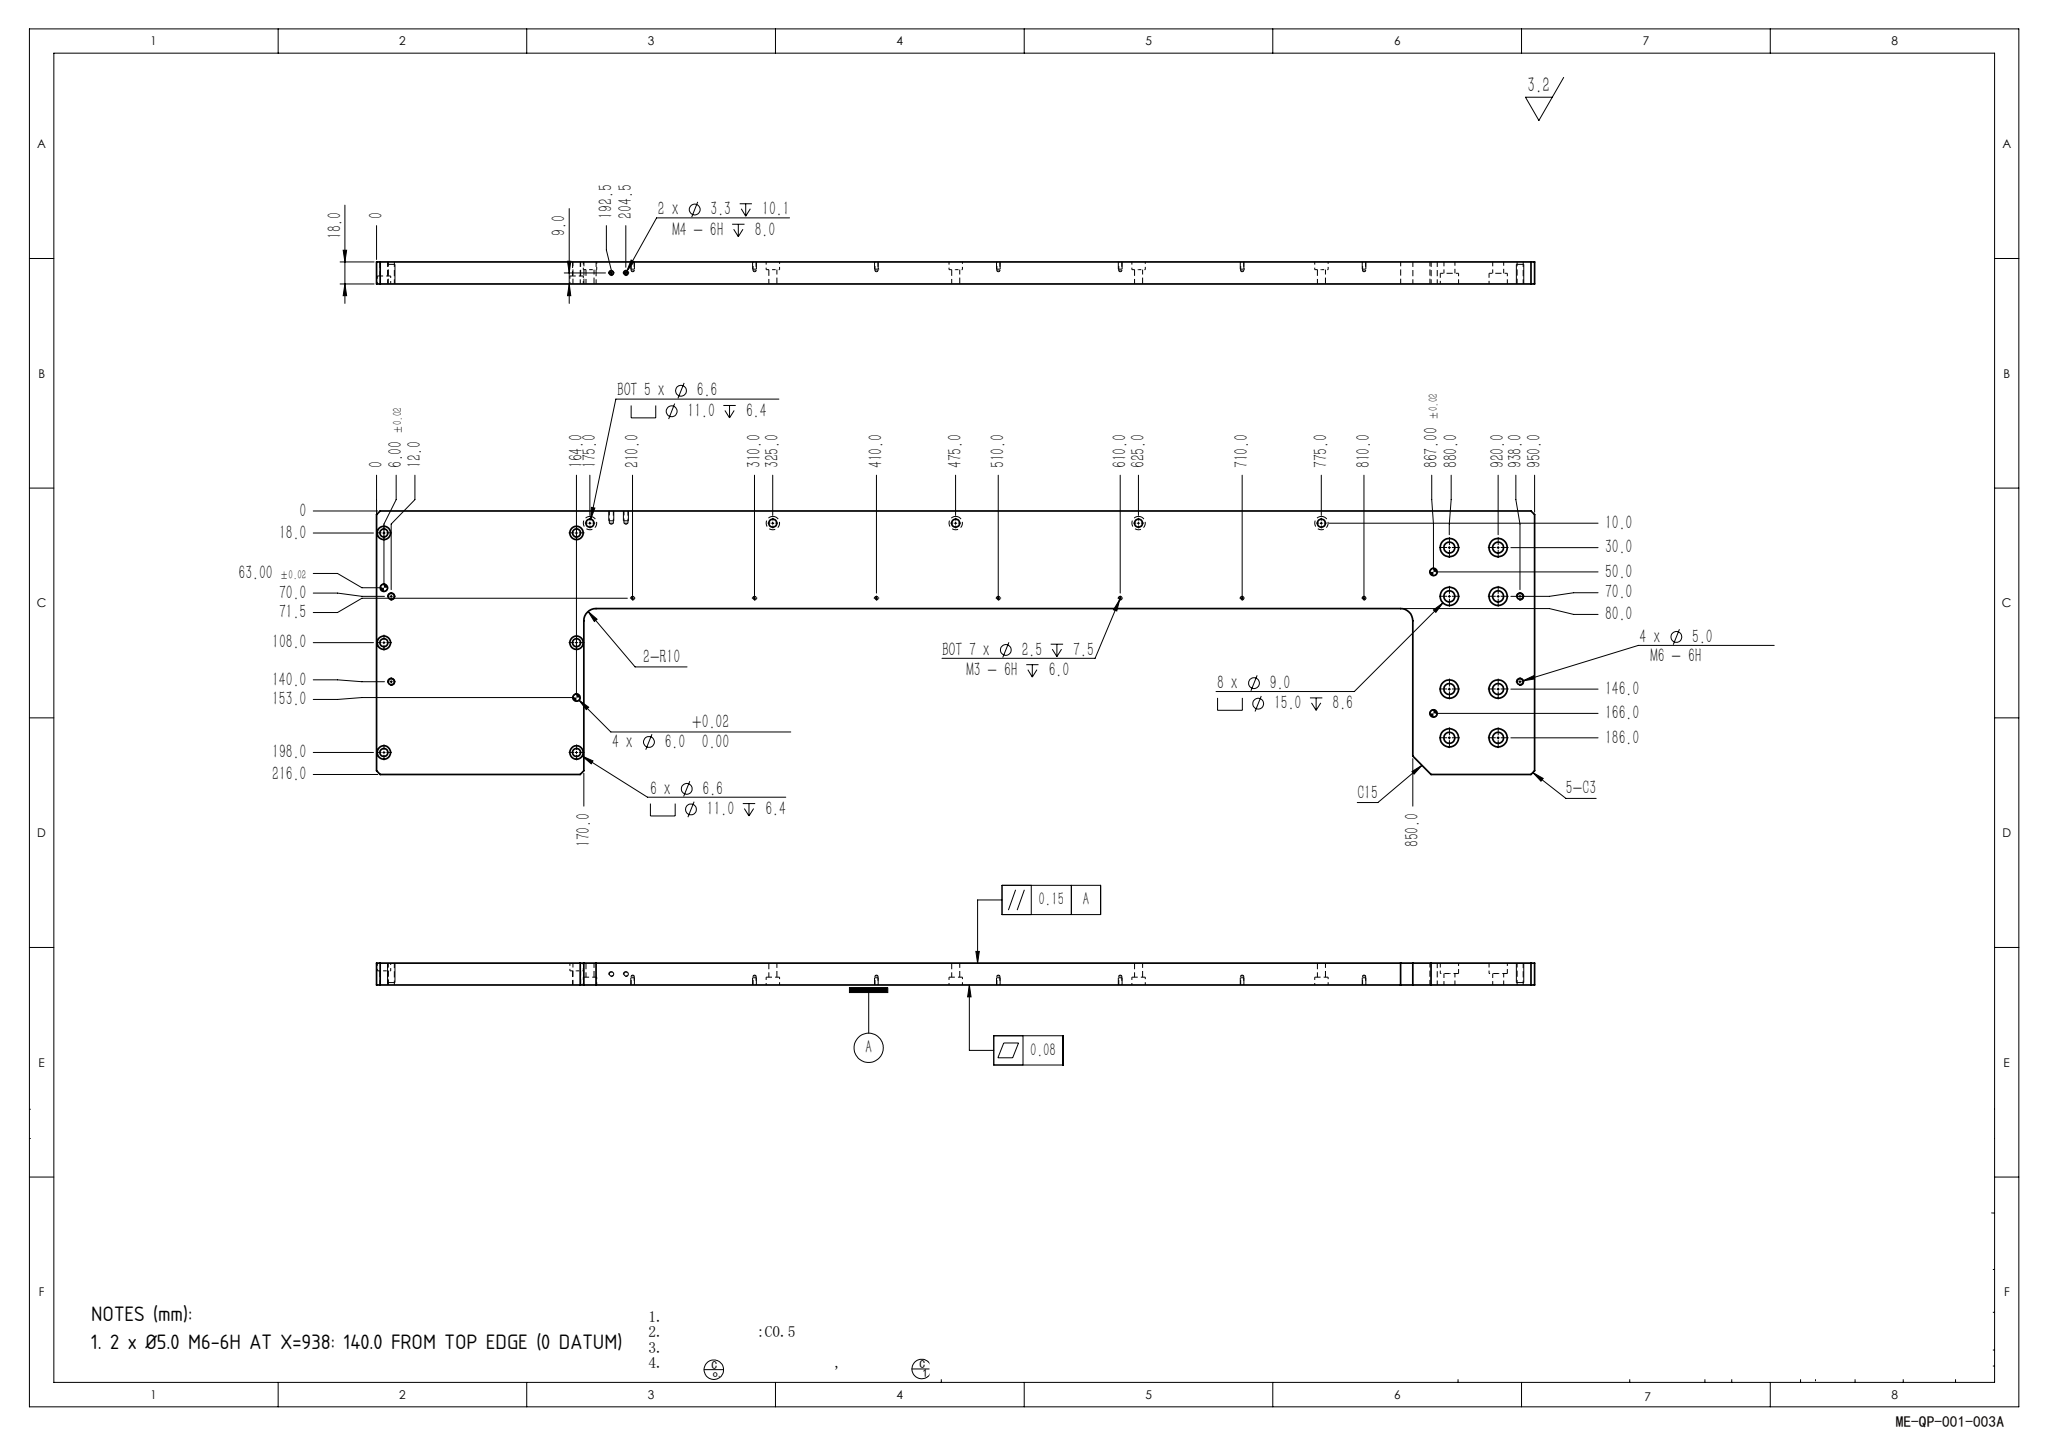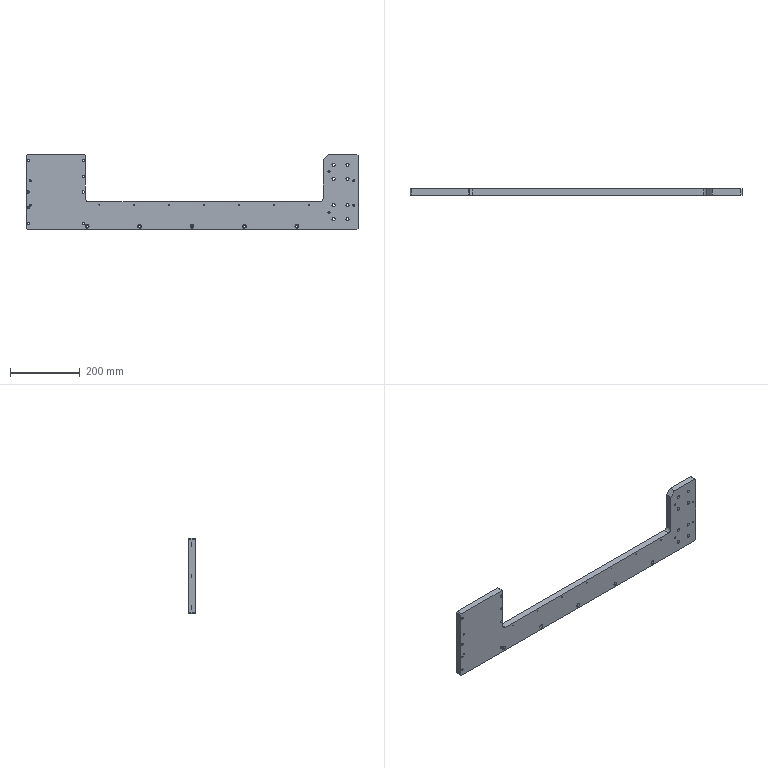Part | SolidWorks | mm | 1 solid | 165 faces | box 950 x 18 x 216 mm | volume 1995411 mm3 | cylinder 112 | plane 35 | cone 18 | commonest cylinder face diameters 11 x22 6.6 x22 15 x16 9 x16 2.5 x14 6 x8 5 x8 3.3 x4
Drawing notes:
2 x Ø5.0 M6-6H AT X=938: 140.0 FROM TOP EDGE (0 DATUM) | from the solid: cylinders [5.0,"y",[938.0,null,140.0],18.0,2] vs [938.0,null,70.0]
build123d program:
from build123d import *

# Parameters (mm, degrees)
BOSS_EXTRUDE1_DEPTH                             = 9
SKETCH14_W                                      = 680
SKETCH14_H                                      = 136
CUT_EXTRUDE2_DEPTH                              = 50
M8_HEX_SOCKET_HEAD_CAP_SCREW_CBORE1_D           = 9
M8_HEX_SOCKET_HEAD_CAP_SCREW_CBORE1_CBORE_D     = 15
M8_HEX_SOCKET_HEAD_CAP_SCREW_CBORE1_CBORE_DEPTH = 8.6
M6_HEX_SOCKET_HEAD_CAP_SCREW_CBORE1_D           = 6.6
M6_HEX_SOCKET_HEAD_CAP_SCREW_CBORE1_CBORE_D     = 11
M6_HEX_SOCKET_HEAD_CAP_SCREW_CBORE1_CBORE_DEPTH = 6.4
SIZE_MM_DOWEL_PIN_HOLE2_D                       = 6
M6_HEX_SOCKET_HEAD_CAP_SCREW_CBORE2_D           = 6.6
M6_HEX_SOCKET_HEAD_CAP_SCREW_CBORE2_CBORE_D     = 11
M6_HEX_SOCKET_HEAD_CAP_SCREW_CBORE2_CBORE_DEPTH = 6.4
M6_TAPPED_HOLE1_D                               = 5
M4_TAPPED_HOLE1_D                               = 3.3
M4_TAPPED_HOLE1_DEPTH                           = 10.1
M4_TAPPED_HOLE1_TIP                             = 0.9914
SIZE_MM_DOWEL_PIN_HOLE3_D                       = 6
M3_TAPPED_HOLE1_D                               = 2.5
M3_TAPPED_HOLE1_DEPTH                           = 7.5
M3_TAPPED_HOLE1_TIP                             = 0.7511
FILLET1_R                                       = 10
CHAMFER1_SIZE                                   = 3
CHAMFER2_SIZE                                   = 15


with BuildPart() as part:
    # Sketch1 → Boss-Extrude1 (new, symmetric)
    with BuildSketch(Plane(origin=(0, 0, 0), x_dir=(1, 0, 0), z_dir=(0, 1, 0))):
        Polygon((375, -90), (-305, -90), (-305, -126), (-475, -126), (-475, -90), (-475, 90), (475, 90), (475, -90), (475, -126), (375, -126), align=None)
    extrude(amount=BOSS_EXTRUDE1_DEPTH, both=True)

    # Sketch14 → Cut-Extrude2 (cut)
    with BuildSketch(Plane.XZ.offset(9)):
        with Locations((35, 58)):
            Rectangle(SKETCH14_W, SKETCH14_H)
    extrude(amount=-CUT_EXTRUDE2_DEPTH, mode=Mode.SUBTRACT)

    # M8 Hex Socket Head Cap Screw CBORE1 (through all)
    with Locations(Plane(origin=(0, 9, 0), x_dir=(1, 0, 0), z_dir=(0, 1, 0))):
        with Locations((405, 60), (445, 60), (405, -96), (445, -96), (405, 20), (445, 20), (405, -56), (445, -56)):
            CounterBoreHole(M8_HEX_SOCKET_HEAD_CAP_SCREW_CBORE1_D / 2, M8_HEX_SOCKET_HEAD_CAP_SCREW_CBORE1_CBORE_D / 2, M8_HEX_SOCKET_HEAD_CAP_SCREW_CBORE1_CBORE_DEPTH)

    # M6 Hex Socket Head Cap Screw CBORE1 (through all)
    with Locations(Plane(origin=(0, 9, 0), x_dir=(1, 0, 0), z_dir=(0, 1, 0))):
        with Locations((-469, -108), (-469, -18), (-469, 72), (-311, 72), (-311, -18), (-311, -108)):
            CounterBoreHole(M6_HEX_SOCKET_HEAD_CAP_SCREW_CBORE1_D / 2, M6_HEX_SOCKET_HEAD_CAP_SCREW_CBORE1_CBORE_D / 2, M6_HEX_SOCKET_HEAD_CAP_SCREW_CBORE1_CBORE_DEPTH)

    # Size mm Dowel Pin Hole2 (through all)
    with Locations(Plane(origin=(0, -9, 0), x_dir=(-1, 0, 0), z_dir=(0, -1, 0))):
        with Locations((469, 27), (311, -63)):
            Hole(SIZE_MM_DOWEL_PIN_HOLE2_D / 2)

    # M6 Hex Socket Head Cap Screw CBORE2 (through all)
    with Locations(Plane(origin=(0, -9, 0), x_dir=(-1, 0, 0), z_dir=(0, -1, 0))):
        with Locations((-300, 80), (-150, 80), (300, 80), (150, 80), (0, 80)):
            CounterBoreHole(M6_HEX_SOCKET_HEAD_CAP_SCREW_CBORE2_D / 2, M6_HEX_SOCKET_HEAD_CAP_SCREW_CBORE2_CBORE_D / 2, M6_HEX_SOCKET_HEAD_CAP_SCREW_CBORE2_CBORE_DEPTH)

    # M6 Tapped Hole1 (through all)
    with Locations(Plane(origin=(0, 9, 0), x_dir=(1, 0, 0), z_dir=(0, 1, 0))):
        with Locations((463, -50), (463, 20), (-463, 20), (-463, -50)):
            Hole(M6_TAPPED_HOLE1_D / 2)

    # M4 Tapped Hole1
    with Locations(Plane(origin=(0, 0, -90), x_dir=(-1, 0, 0), z_dir=(0, 0, -1))):
        with Locations((270.5, 0), (282.5, 0)):
            Hole(M4_TAPPED_HOLE1_D / 2, depth=M4_TAPPED_HOLE1_DEPTH)
            with Locations((0, 0, -(M4_TAPPED_HOLE1_DEPTH + M4_TAPPED_HOLE1_TIP / 2))):  # 118° drill point
                Cone(0, M4_TAPPED_HOLE1_D / 2, M4_TAPPED_HOLE1_TIP, mode=Mode.SUBTRACT)

    # Size mm Dowel Pin Hole3 (through all)
    with Locations(Plane(origin=(0, -9, 0), x_dir=(-1, 0, 0), z_dir=(0, -1, 0))):
        with Locations((-392, 40), (-392, -76)):
            Hole(SIZE_MM_DOWEL_PIN_HOLE3_D / 2)

    # M3 Tapped Hole1
    with Locations(Plane(origin=(0, -9, 0), x_dir=(-1, 0, 0), z_dir=(0, -1, 0))):
        with Locations((265, 18.5), (165, 18.5), (65, 18.5), (-35, 18.5), (-135, 18.5), (-235, 18.5), (-335, 18.5)):
            Hole(M3_TAPPED_HOLE1_D / 2, depth=M3_TAPPED_HOLE1_DEPTH)
            with Locations((0, 0, -(M3_TAPPED_HOLE1_DEPTH + M3_TAPPED_HOLE1_TIP / 2))):  # 118° drill point
                Cone(0, M3_TAPPED_HOLE1_D / 2, M3_TAPPED_HOLE1_TIP, mode=Mode.SUBTRACT)

    # Fillet1
    fillet1_edges = [part.edges().sort_by_distance(p)[0] for p in [
        (-305, 0, -10),
        (375, 0, -10),
    ]]
    fillet(fillet1_edges, radius=FILLET1_R)

    # Chamfer1
    chamfer1_edges = [part.edges().sort_by_distance(p)[0] for p in [
        (-475, 0, -90),
        (475, 0, -90),
        (475, 0, 126),
        (-305, 0, 126),
        (-475, 0, 126),
    ]]
    chamfer(chamfer1_edges, length=CHAMFER1_SIZE)

    # Chamfer2
    chamfer2_edges = [part.edges().sort_by_distance(p)[0] for p in [
        (375, 0, 126),
    ]]
    chamfer(chamfer2_edges, length=CHAMFER2_SIZE)


solid = part.part